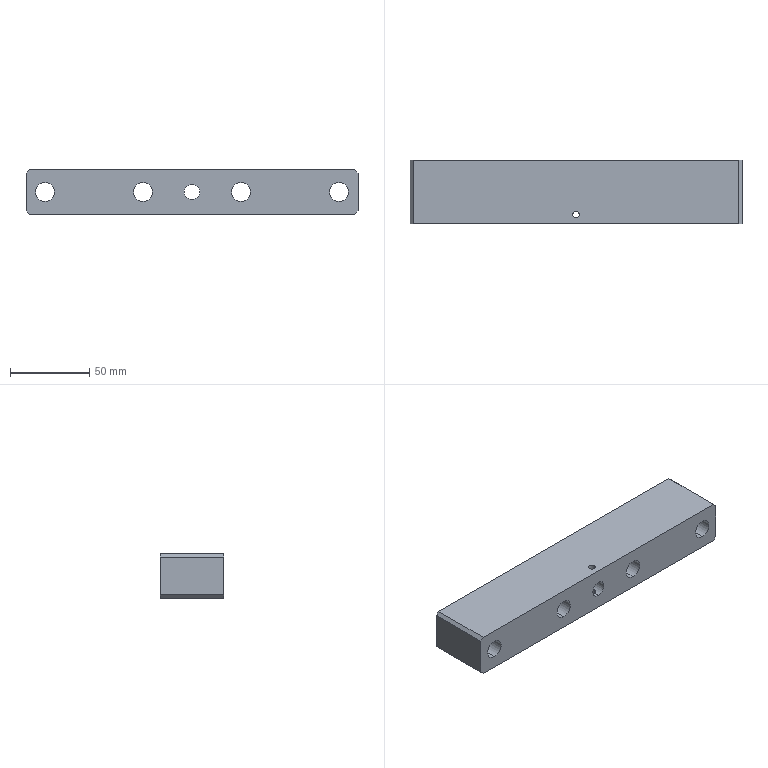Component | SolidWorks | 04LowerMaterialReceivingSwingAngleAssembly(3920)-1_H2020022-0449-1(3920)-2 | 1 solid | 84 faces | box 210 x 40 x 28 mm | volume 211916 mm3 | cylinder 46 | cone 24 | plane 14 | commonest cylinder face diameters 2.5 x24 15 x8 12 x8 4.2 x4 10 x2 | material 6061 Aluminum Alloy
build123d program:
from build123d import *

# Parameters (mm, degrees)
SKETCH1_W           = 210
SKETCH1_H           = 28
BOSS_EXTRUDE1_DEPTH = 40
SKETCH2_R           = 6
CUT_EXTRUDE1_DEPTH  = 216.601
SKETCH3_R           = 7.5
CUT_EXTRUDE3_DEPTH  = 4
CIRPATTERN1_COUNT   = 3
LPATTERN1_COUNT     = 4
LPATTERN1_PITCH     = 62
CHAMFER1_SIZE       = 2
SKETCH8_R           = 5
CUT_EXTRUDE6_DEPTH  = 216.601
M5_TAPPED_HOLE1_D   = 4.2


with BuildPart() as part:
    # Sketch1 → Boss-Extrude1 (new body)
    with BuildSketch(Plane(origin=(0, 0, 0), x_dir=(1, 0, 0), z_dir=(0, 1, 0))):
        with Locations((105, -14)):
            Rectangle(SKETCH1_W, SKETCH1_H)
    extrude(amount=BOSS_EXTRUDE1_DEPTH)

    # Sketch2 → Cut-Extrude1 (cut, through all)
    with BuildSketch(Plane(origin=(0, 40, 0), x_dir=(1, 0, 0), z_dir=(0, 1, 0))):
        with Locations(Location((12, -14, 0), (0, 0, 270))):
            Circle(SKETCH2_R)
    cut_extrude1 = extrude(amount=-CUT_EXTRUDE1_DEPTH, mode=Mode.SUBTRACT)

    # Sketch3 → Cut-Extrude3 (cut)
    with BuildSketch(Plane.XZ):
        with Locations(Location((12, 14, 0), (0, 0, 270))):
            Circle(SKETCH3_R)
    cut_extrude3 = extrude(amount=-CUT_EXTRUDE3_DEPTH, mode=Mode.SUBTRACT)

    # Sketch5 → M3 Tapped Hole1 (revolve, cut)
    with BuildSketch(Plane(origin=(3, 0, 14), x_dir=(0, 0, -1), z_dir=(1, 0, 0))):
        Polygon((0, 0), (0, 8.251), (1.25, 7.5), (1.25, 0), align=None)
    m3_tapped_hole1 = revolve(axis=Axis((3, -6.35, 14), (0, 1, 0)), mode=Mode.SUBTRACT)

    # CirPattern1: M3 Tapped Hole1 ×3 about axis
    cirpattern1_axis = Axis((12, 0, 14), (0, 1, 0))
    for i in range(1, CIRPATTERN1_COUNT):
        add(m3_tapped_hole1.rotate(cirpattern1_axis, i * 360 / CIRPATTERN1_COUNT), mode=Mode.SUBTRACT)

    # LPattern1: Cut-Extrude1, Cut-Extrude3, M3 Tapped Hole1 ×4
    with Locations(*[(i * LPATTERN1_PITCH, 0, 0) for i in range(1, LPATTERN1_COUNT)]):
        add(cut_extrude1, mode=Mode.SUBTRACT)
        add(cut_extrude3, mode=Mode.SUBTRACT)
        add(m3_tapped_hole1, mode=Mode.SUBTRACT)

    # LPattern1 copy 1 sketch → LPattern1 copy 1 (revolve, cut)
    with BuildSketch(Plane(origin=(78.5, 0, 21.794), x_dir=(-0.866, 0, 0.5), z_dir=(-0.5, 0, -0.866))):
        Polygon((0, 0), (0, 8.251), (1.25, 7.5), (1.25, 0), align=None)
    revolve(axis=Axis((78.5, -6.35, 21.794), (0, 1, 0)), mode=Mode.SUBTRACT)

    # LPattern1 copy 2 sketch → LPattern1 copy 2 (revolve, cut)
    with BuildSketch(Plane(origin=(140.5, 0, 21.794), x_dir=(-0.866, 0, 0.5), z_dir=(-0.5, 0, -0.866))):
        Polygon((0, 0), (0, 8.251), (1.25, 7.5), (1.25, 0), align=None)
    revolve(axis=Axis((140.5, -6.35, 21.794), (0, 1, 0)), mode=Mode.SUBTRACT)

    # LPattern1 copy 3 sketch → LPattern1 copy 3 (revolve, cut)
    with BuildSketch(Plane(origin=(202.5, 0, 21.794), x_dir=(-0.866, 0, 0.5), z_dir=(-0.5, 0, -0.866))):
        Polygon((0, 0), (0, 8.251), (1.25, 7.5), (1.25, 0), align=None)
    revolve(axis=Axis((202.5, -6.35, 21.794), (0, 1, 0)), mode=Mode.SUBTRACT)

    # LPattern1 copy 4 sketch → LPattern1 copy 4 (revolve, cut)
    with BuildSketch(Plane(origin=(78.5, 0, 6.206), x_dir=(0.866, 0, 0.5), z_dir=(-0.5, 0, 0.866))):
        Polygon((0, 0), (0, 8.251), (1.25, 7.5), (1.25, 0), align=None)
    revolve(axis=Axis((78.5, -6.35, 6.206), (0, 1, 0)), mode=Mode.SUBTRACT)

    # LPattern1 copy 5 sketch → LPattern1 copy 5 (revolve, cut)
    with BuildSketch(Plane(origin=(140.5, 0, 6.206), x_dir=(0.866, 0, 0.5), z_dir=(-0.5, 0, 0.866))):
        Polygon((0, 0), (0, 8.251), (1.25, 7.5), (1.25, 0), align=None)
    revolve(axis=Axis((140.5, -6.35, 6.206), (0, 1, 0)), mode=Mode.SUBTRACT)

    # LPattern1 copy 6 sketch → LPattern1 copy 6 (revolve, cut)
    with BuildSketch(Plane(origin=(202.5, 0, 6.206), x_dir=(0.866, 0, 0.5), z_dir=(-0.5, 0, 0.866))):
        Polygon((0, 0), (0, 8.251), (1.25, 7.5), (1.25, 0), align=None)
    revolve(axis=Axis((202.5, -6.35, 6.206), (0, 1, 0)), mode=Mode.SUBTRACT)

    # Chamfer1
    chamfer1_edges = [part.edges().sort_by_distance(p)[0] for p in [
        (0, 20, 0),
        (210, 20, 0),
        (210, 20, 28),
        (0, 20, 28),
    ]]
    chamfer(chamfer1_edges, length=CHAMFER1_SIZE)

    # Sketch8 → Cut-Extrude6 (cut, through all)
    with BuildSketch(Plane(origin=(0, 40, 0), x_dir=(1, 0, 0), z_dir=(0, 1, 0))):
        with Locations(Location((105, -14, 0), (0, 0, 270))):
            Circle(SKETCH8_R)
    extrude(amount=-CUT_EXTRUDE6_DEPTH, mode=Mode.SUBTRACT)

    # M5 Tapped Hole1 (through all)
    with Locations(Plane.XY.offset(28)):
        with Locations((105, 34.25)):
            Hole(M5_TAPPED_HOLE1_D / 2)


solid = part.part

# Placed as in the assembly
solid = solid.moved(Location((-135.964, 171.813, 294.197), (180, 0, 0)))